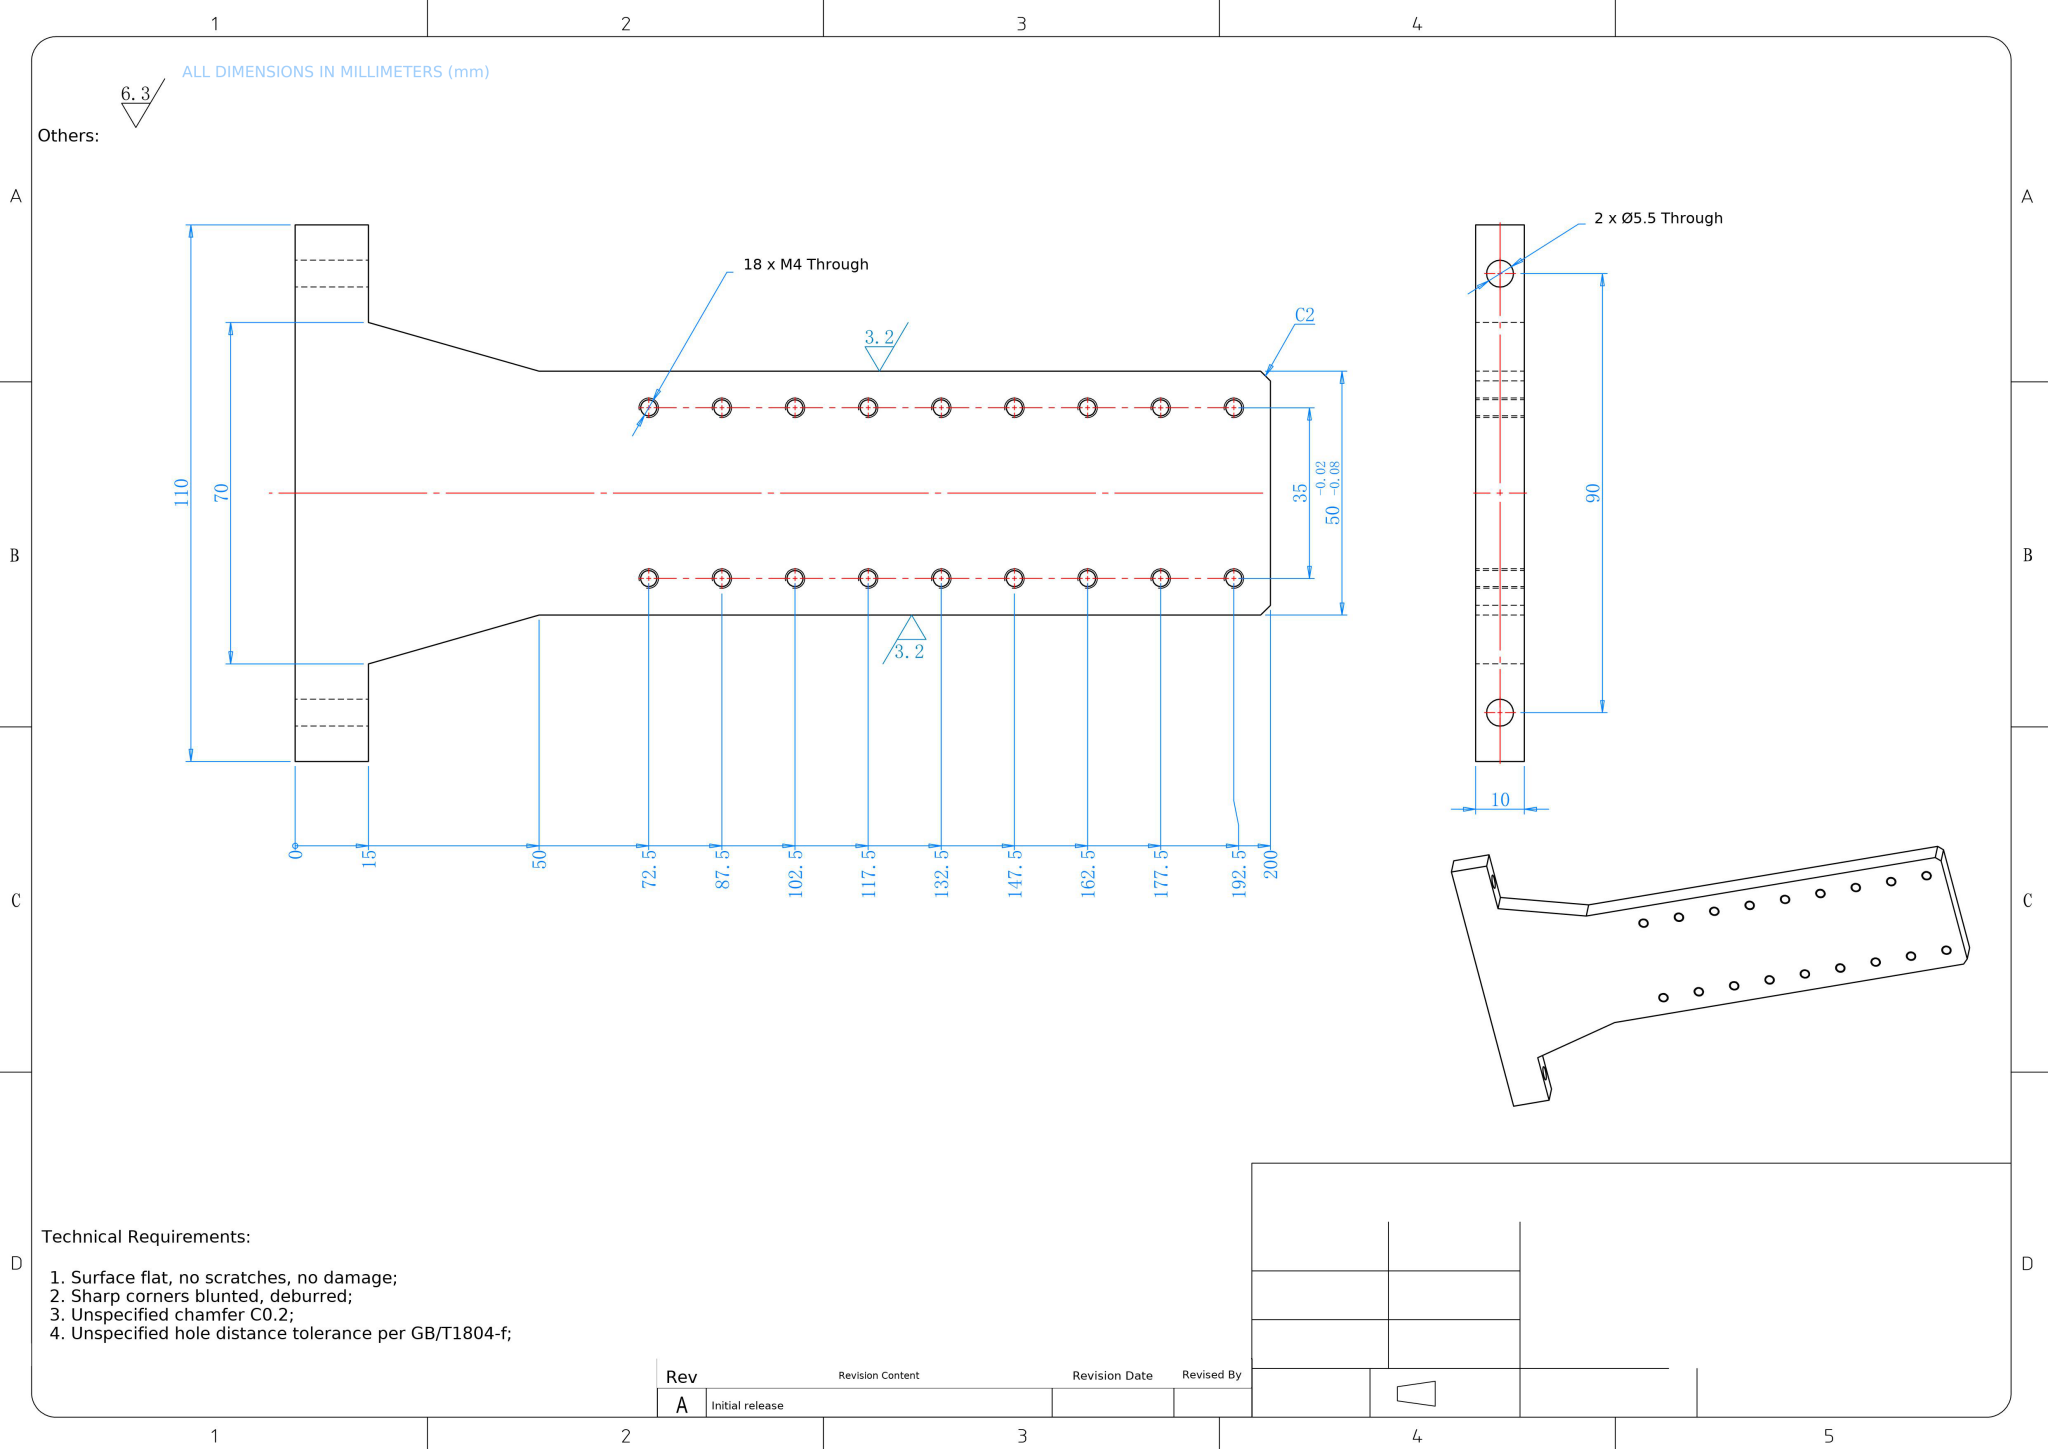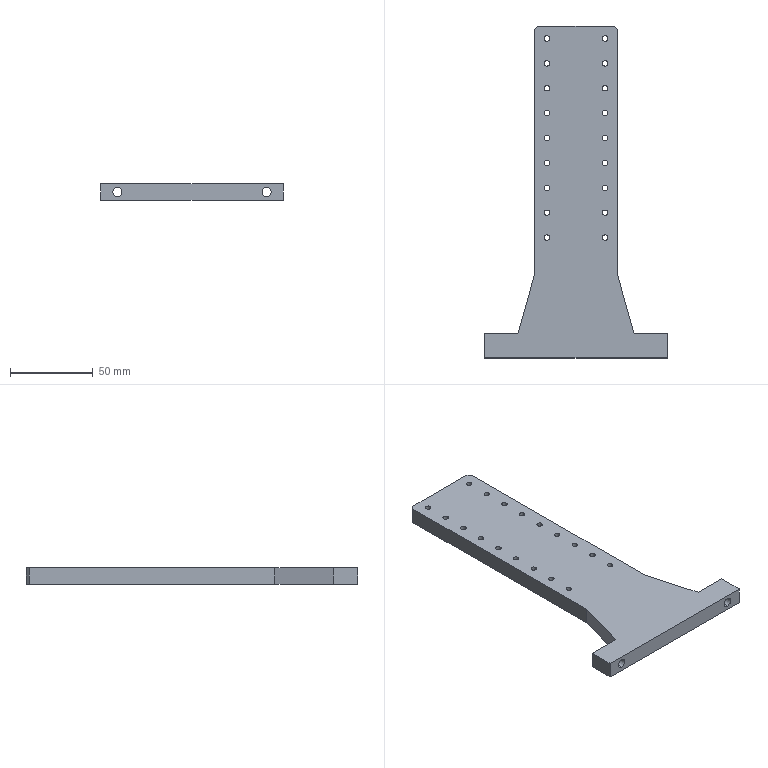Part | NX | mm | 1 solid | 54 faces | box 110 x 200 x 10 mm | volume 110208 mm3 | cylinder 40 | plane 14 | commonest cylinder face diameters 3.3 x36 5.5 x4